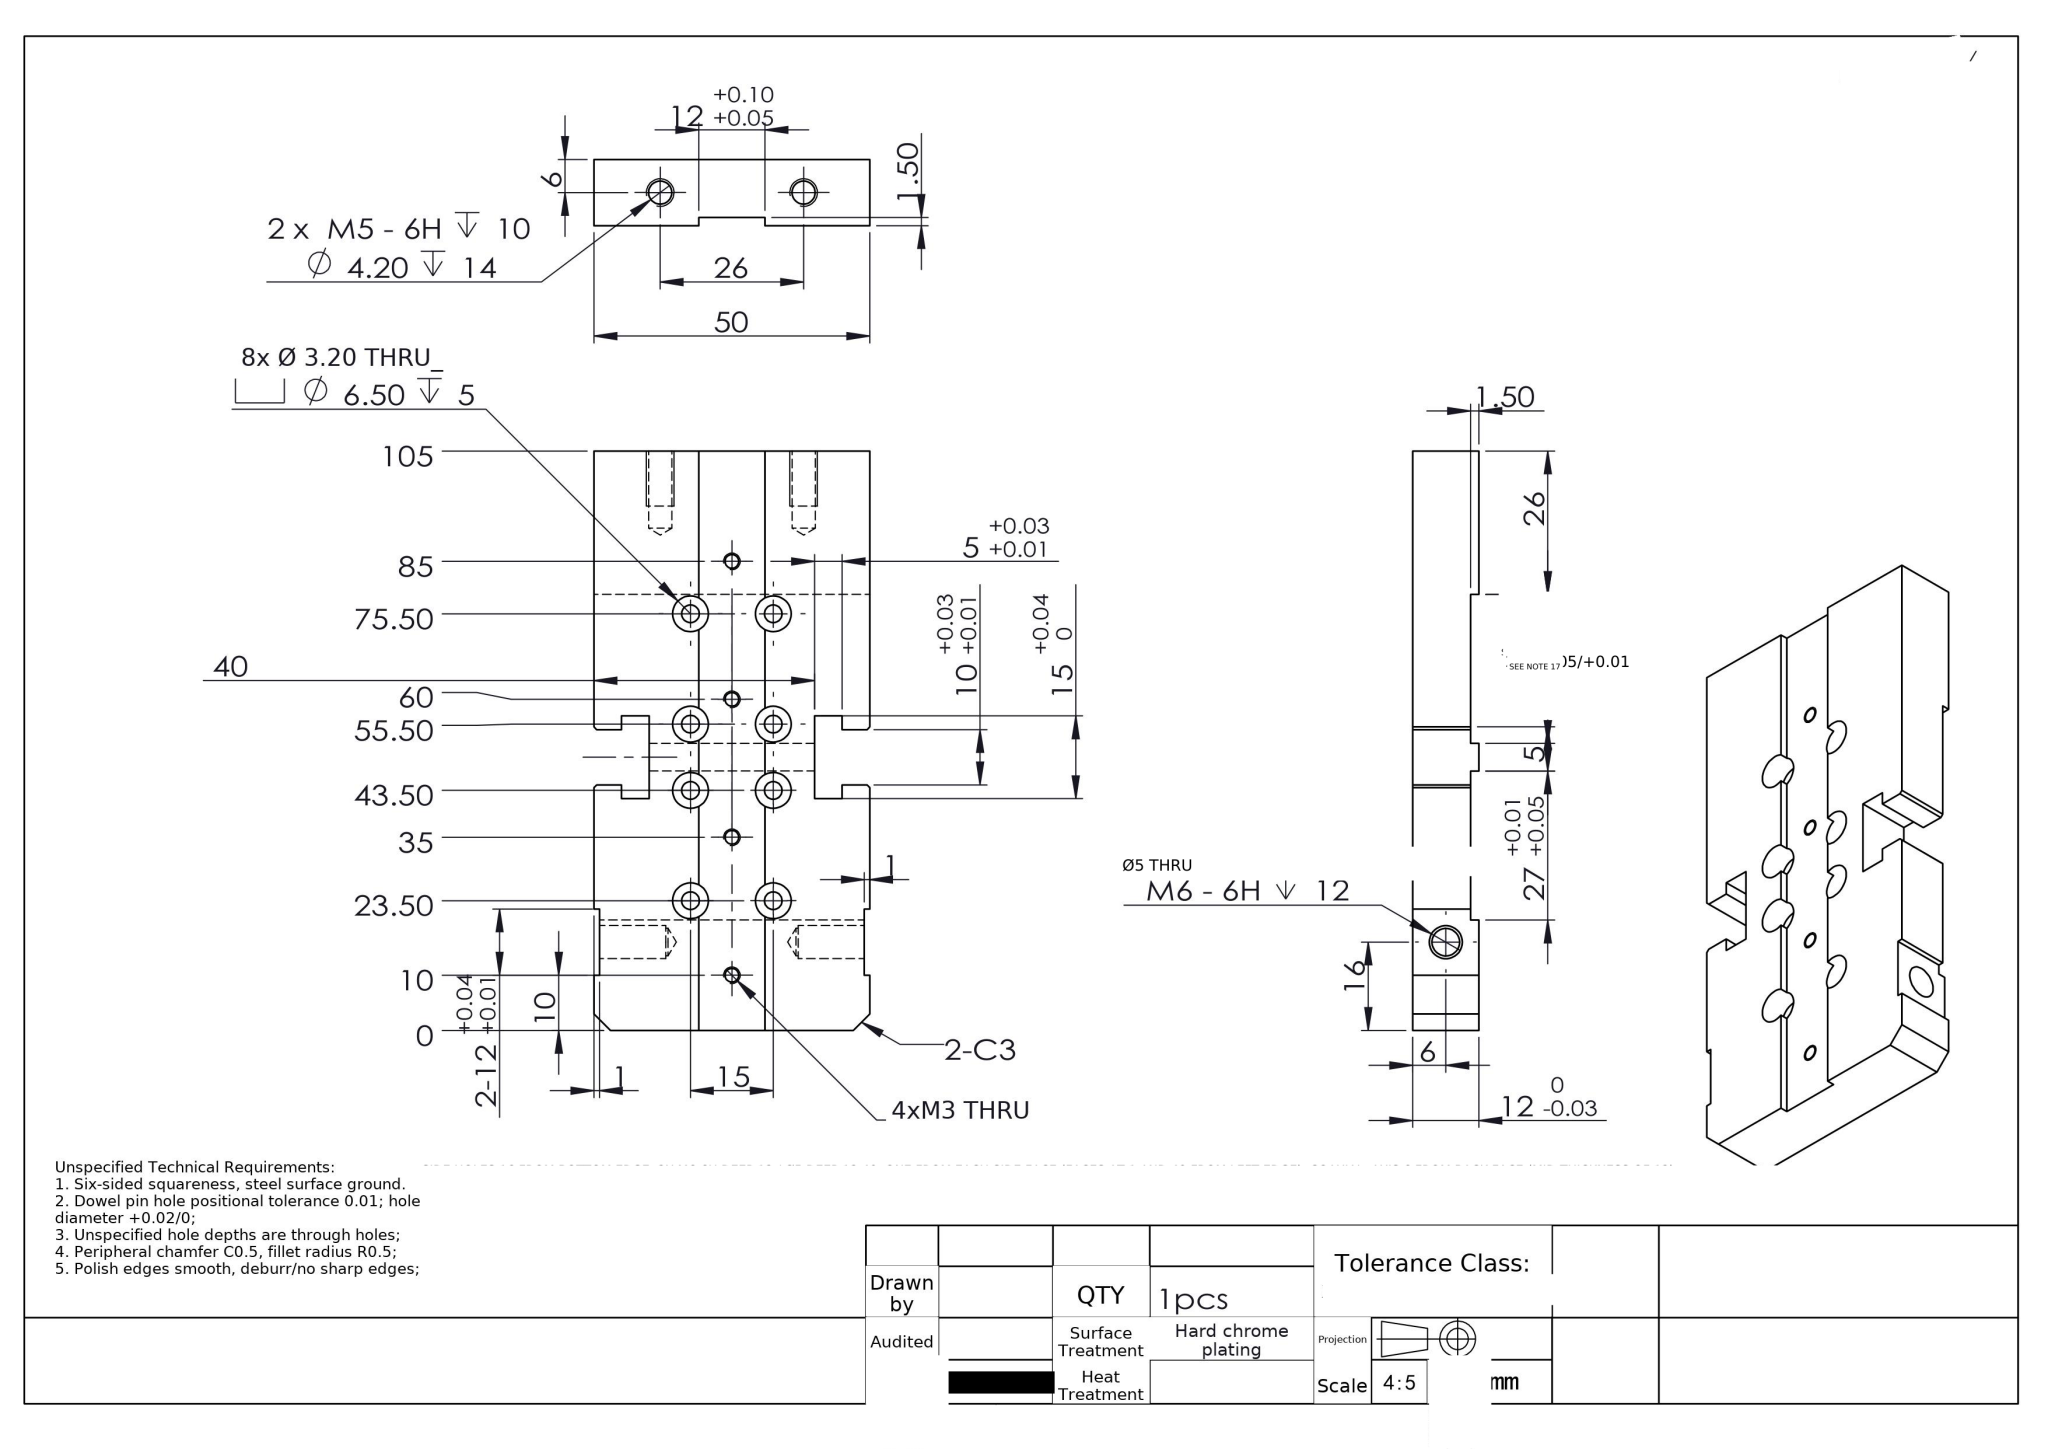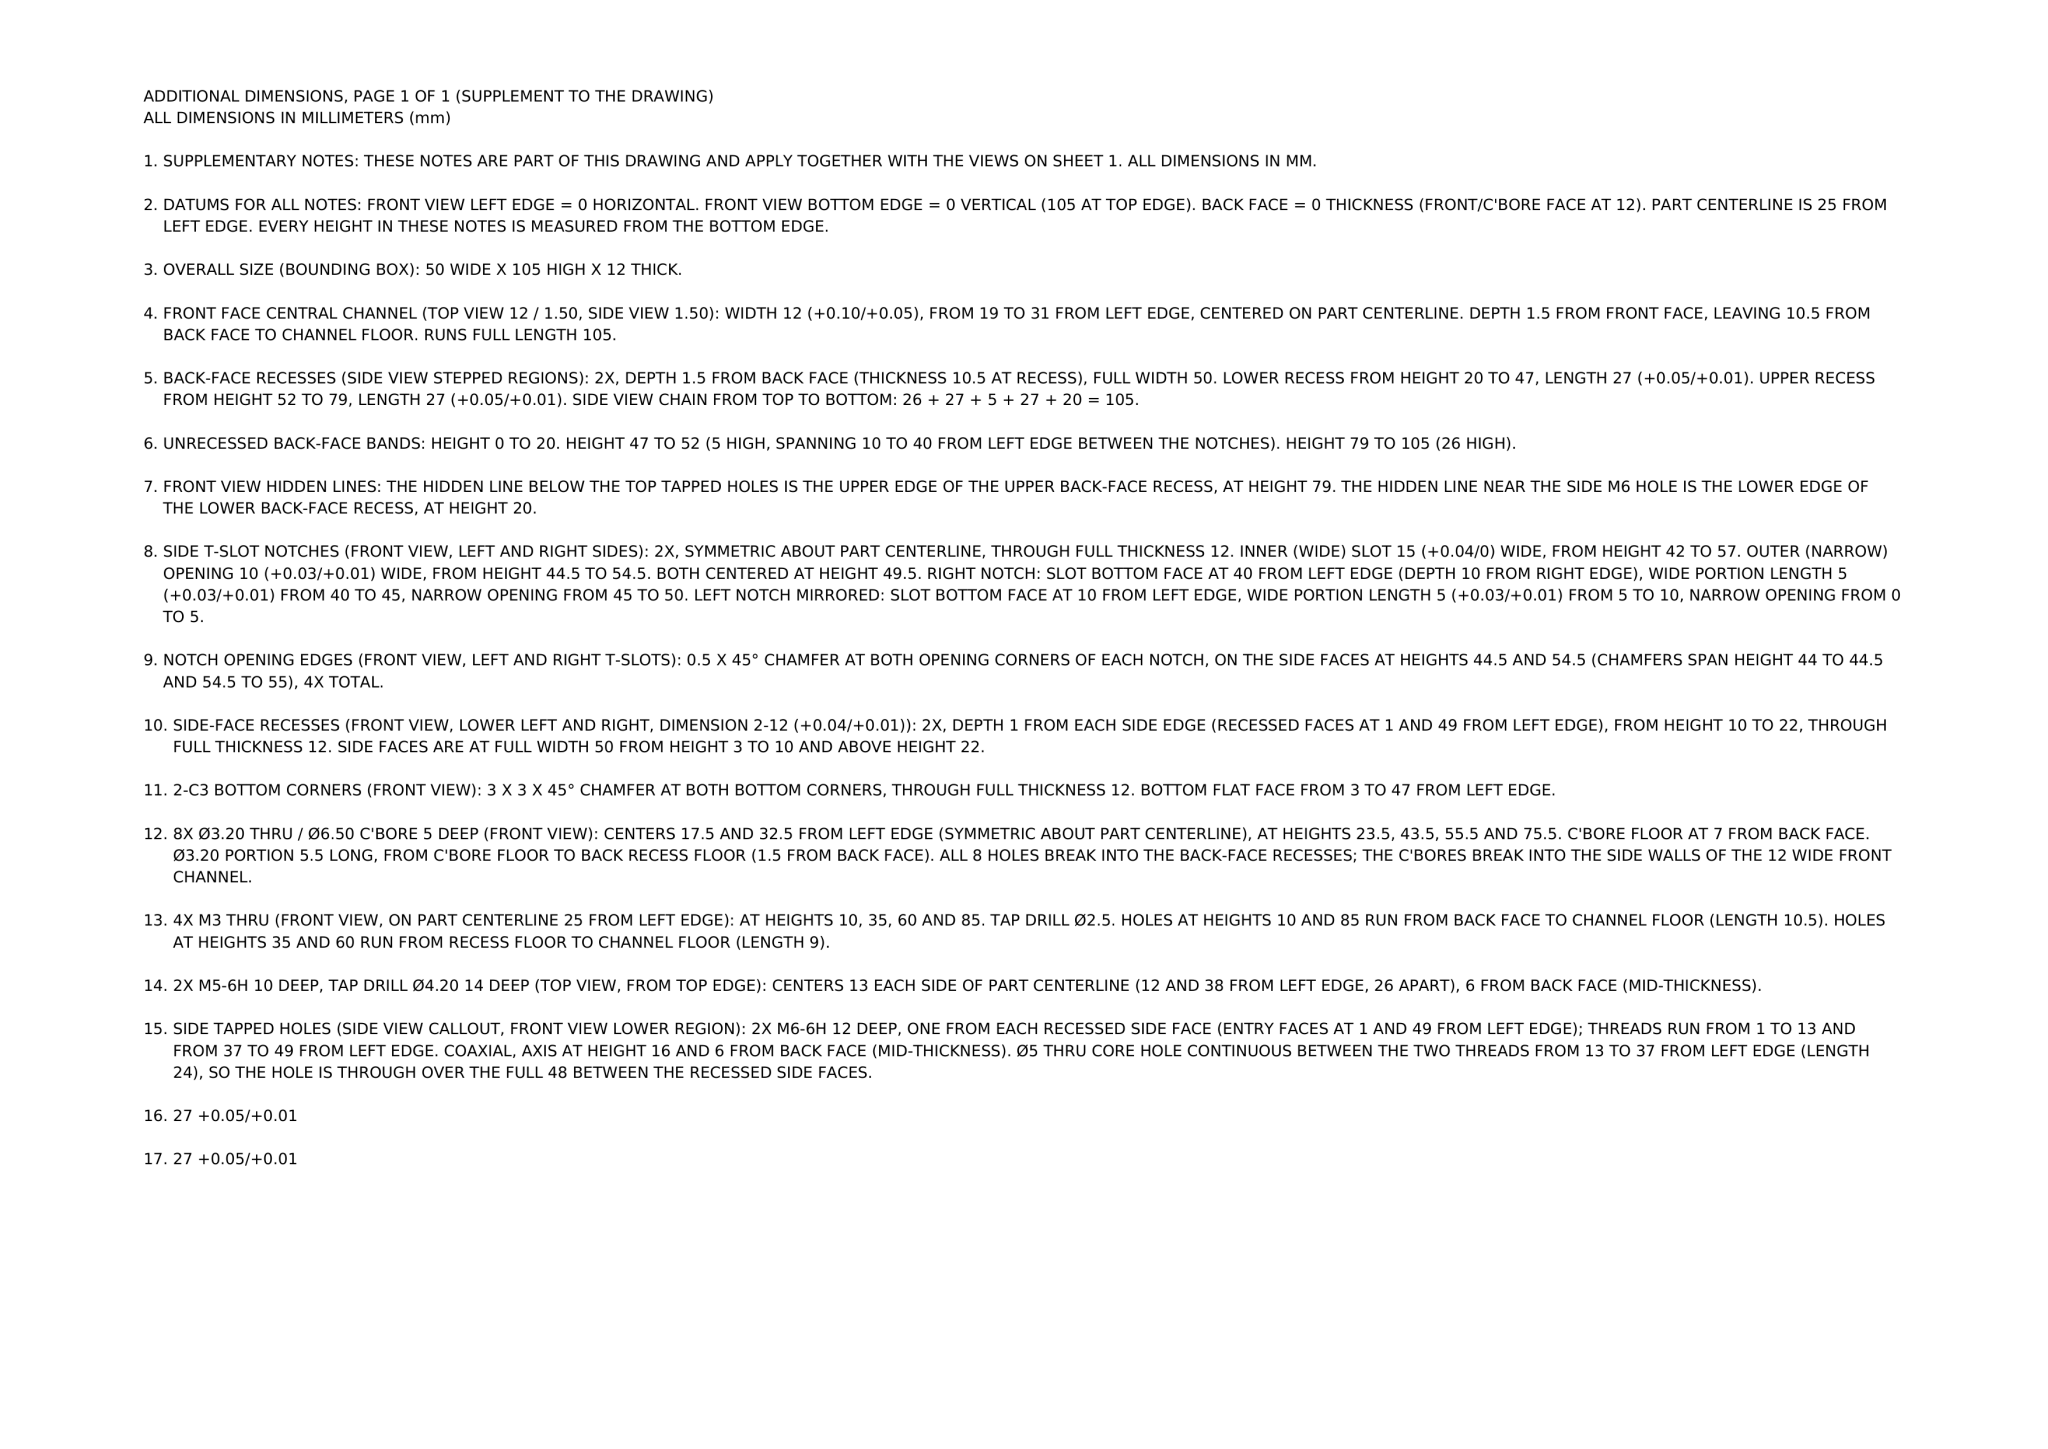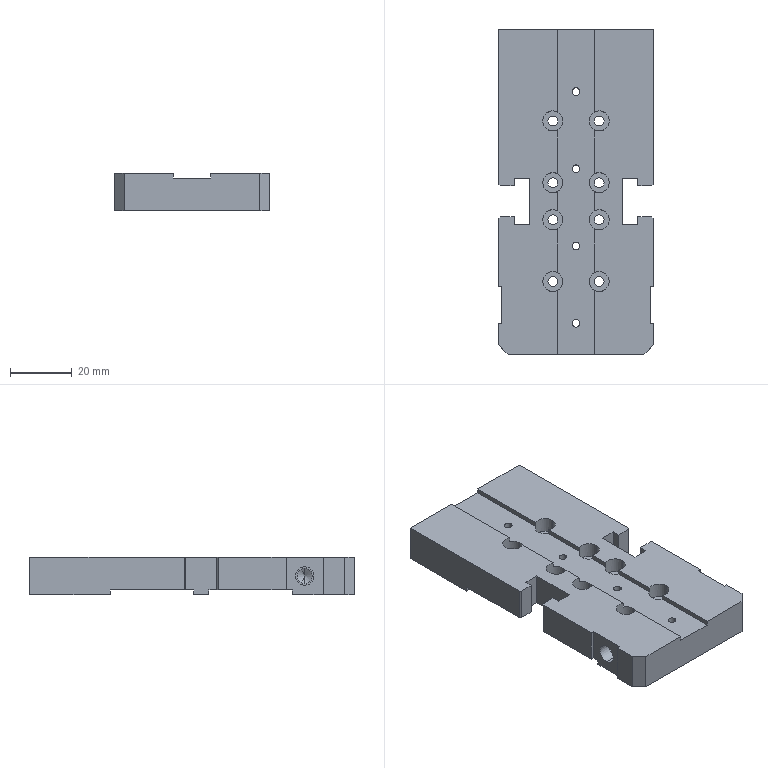Part | NX | mm | 1 solid | 126 faces | box 50 x 105 x 12 mm | volume 50990 mm3 | plane 66 | cylinder 52 | cone 8 | commonest cylinder face diameters 6.5 x16 3.2 x16 2.5 x8 6 x4 5 x4 4.2 x4